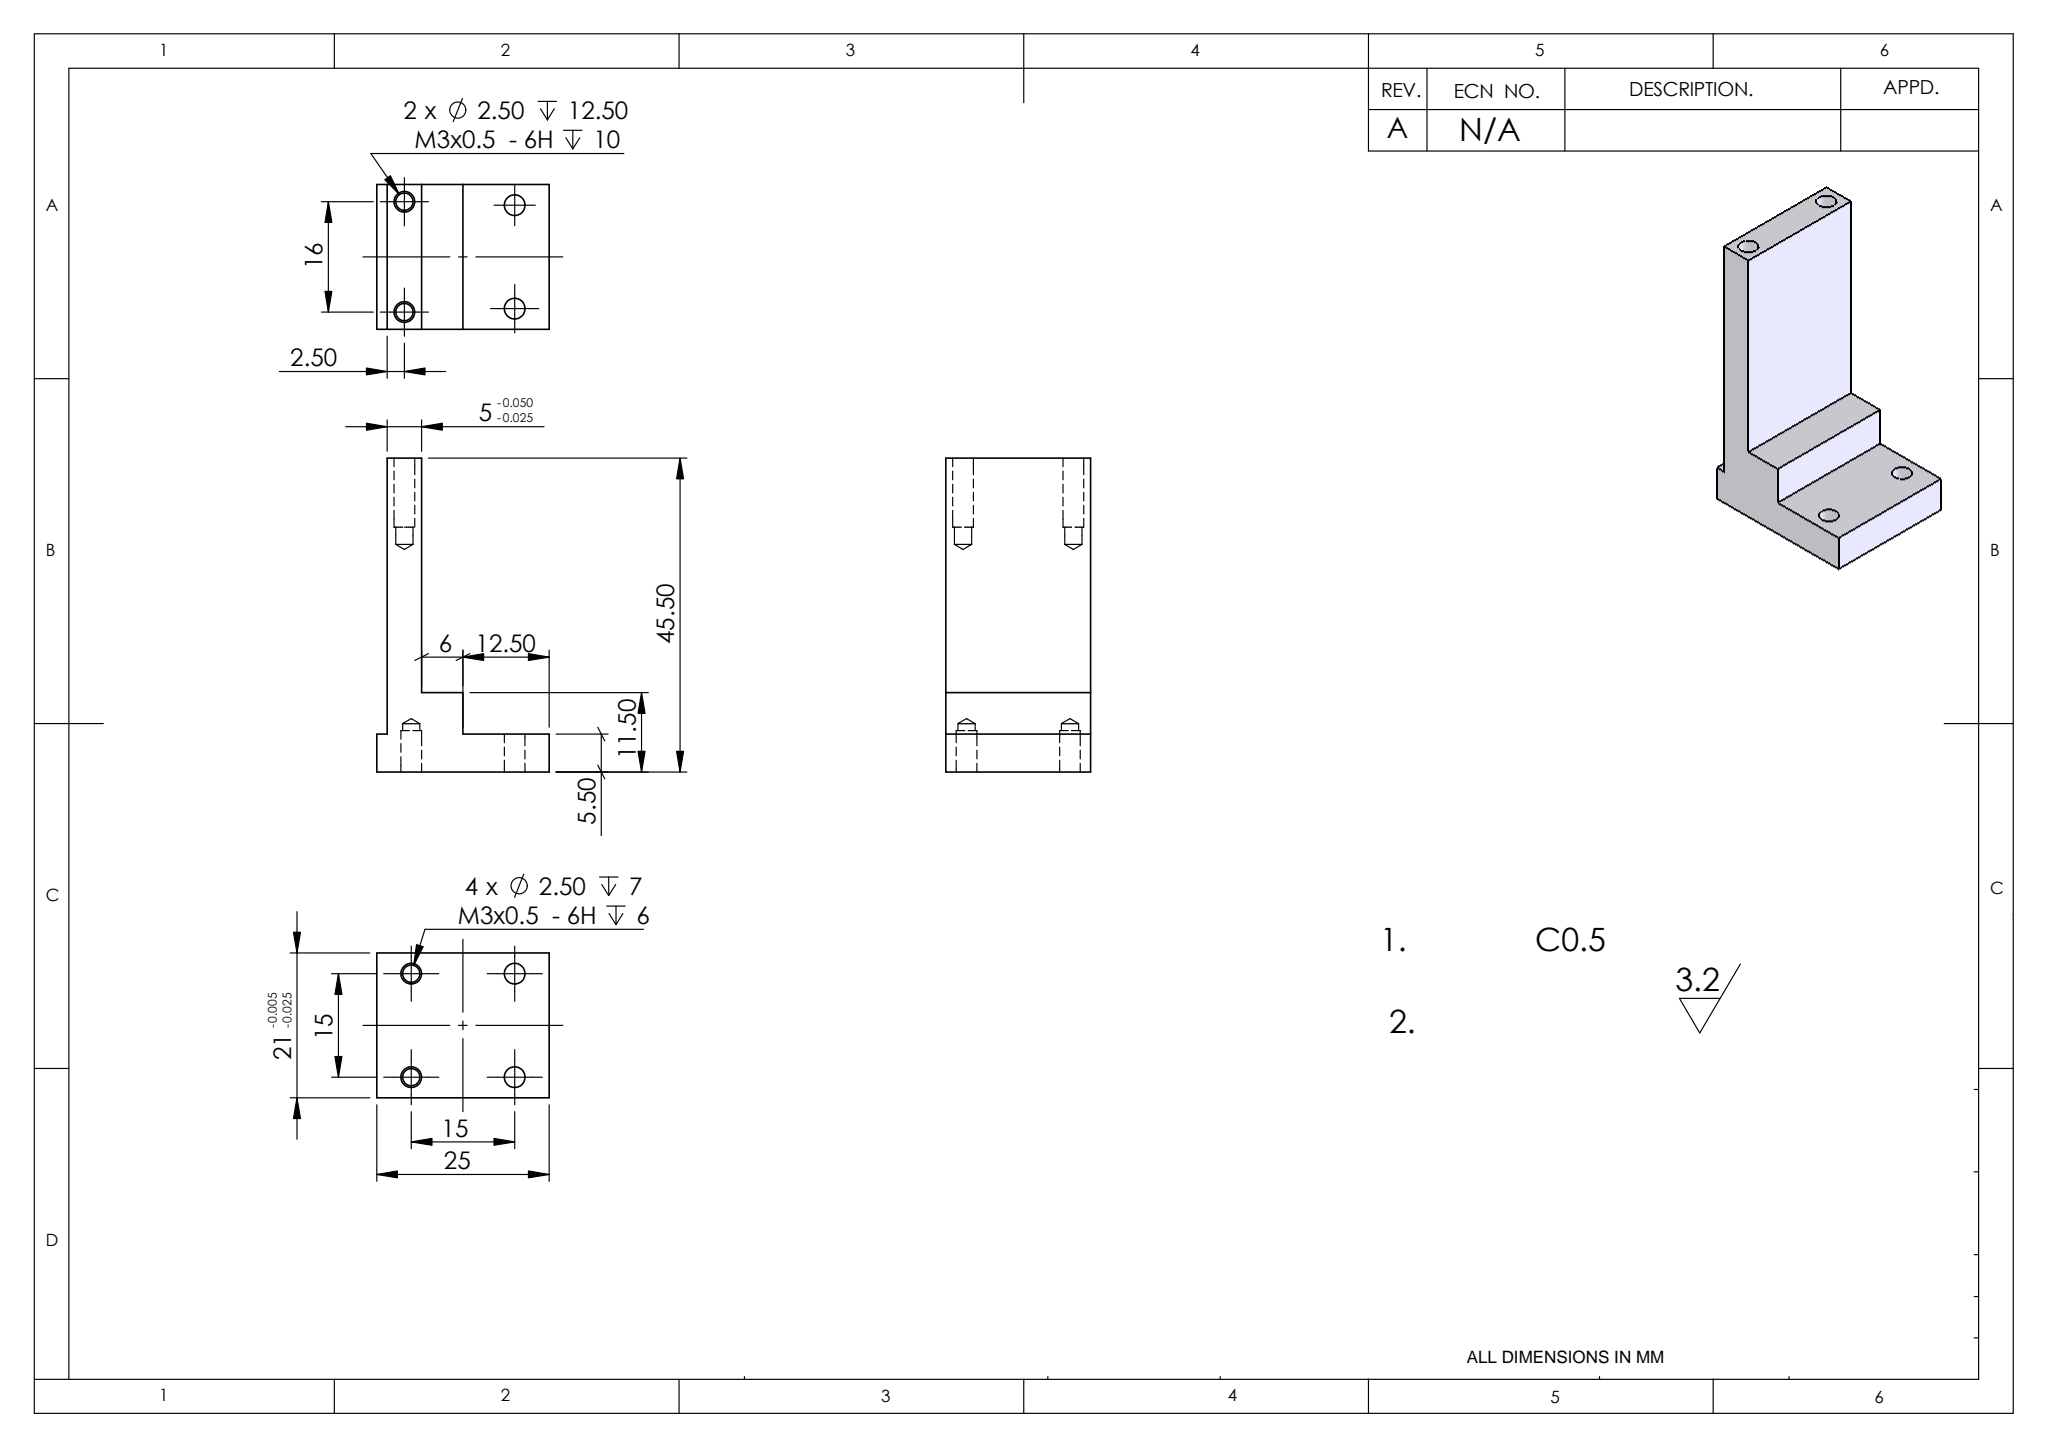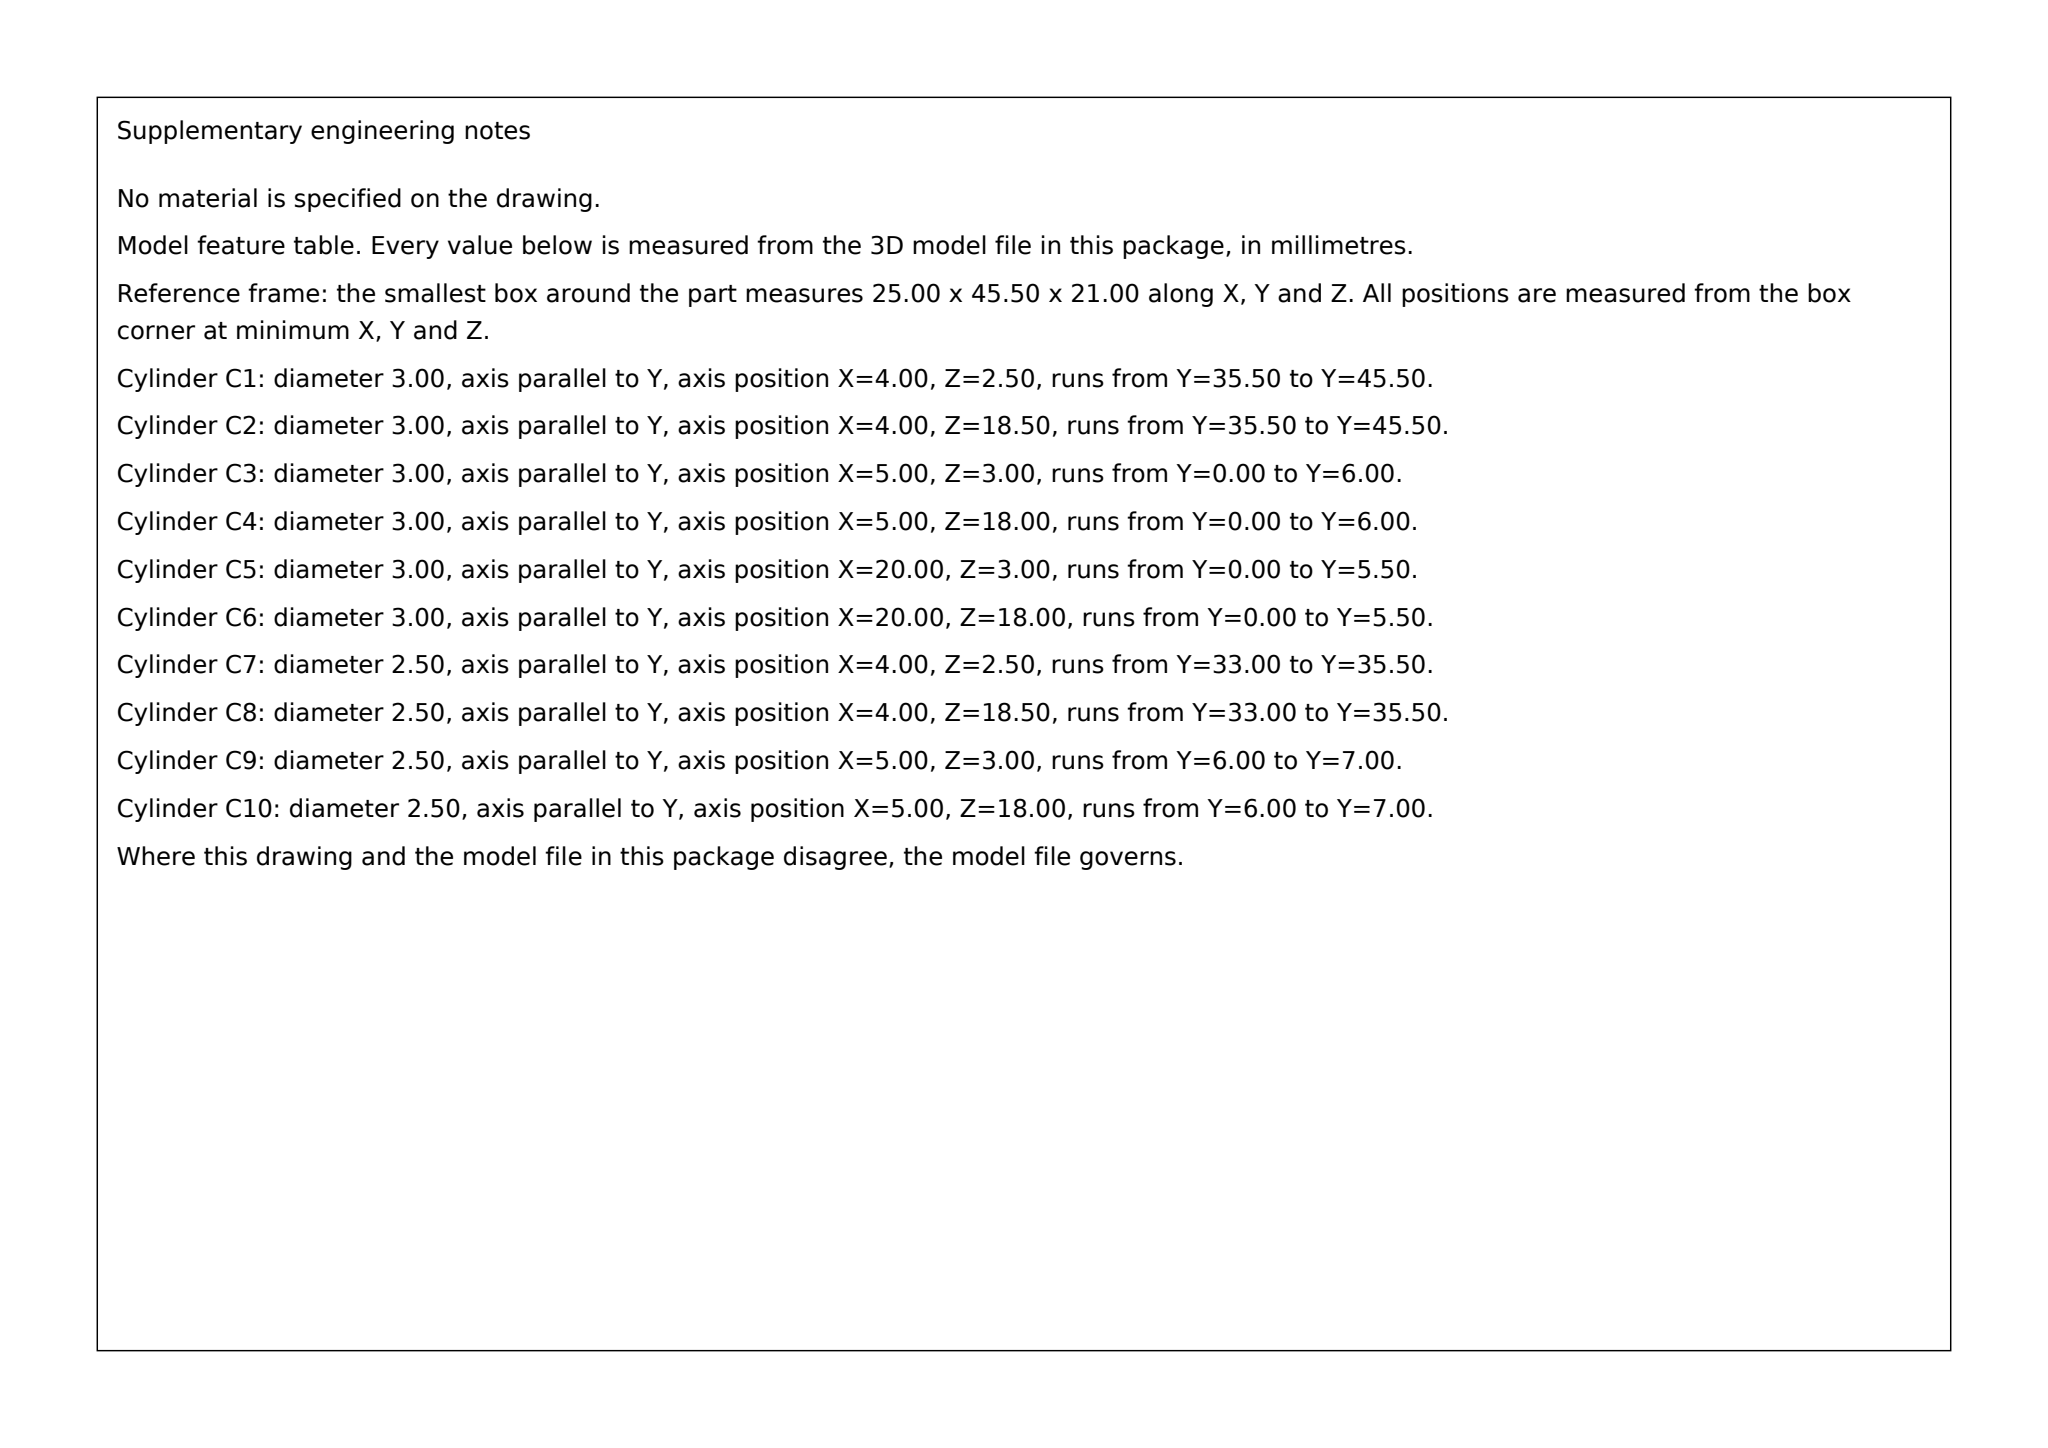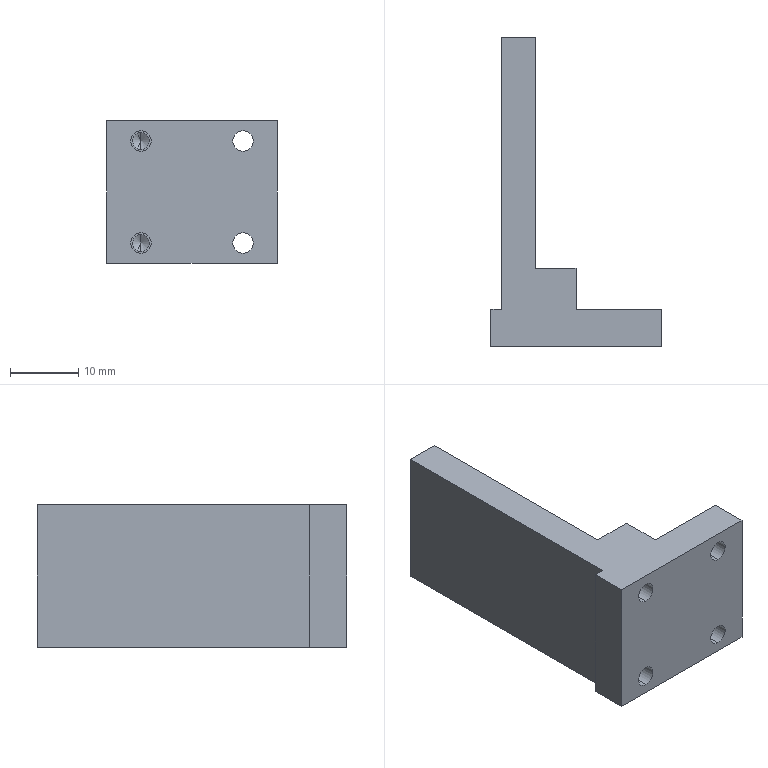Part | SolidWorks | mm | 1 solid | 44 faces | box 25 x 45.5 x 21 mm | volume 7500 mm3 | cylinder 20 | plane 16 | cone 8 | commonest cylinder face diameters 3 x12 2.5 x8
build123d program:
from build123d import *

# Parameters (mm, degrees)
SKETCH2_W                   = 21
SKETCH2_H                   = 40
EXTRUDE1_DEPTH              = 5
M3_TAPPED_HOLE1_D           = 2.5
M3_TAPPED_HOLE1_DEPTH       = 12.5
M3_TAPPED_HOLE1_CBORE_D     = 3
M3_TAPPED_HOLE1_CBORE_DEPTH = 10
M3_TAPPED_HOLE1_TIP         = 0.7511
SKETCH5_W                   = 25
SKETCH5_H                   = 21
EXTRUDE2_DEPTH              = 5.5
SKETCH8_W                   = 6
SKETCH8_H                   = 6
EXTRUDE3_DEPTH              = 21
M3_TAPPED_HOLE2_D           = 2.5
M3_TAPPED_HOLE2_DEPTH       = 7
M3_TAPPED_HOLE2_CBORE_D     = 3
M3_TAPPED_HOLE2_CBORE_DEPTH = 6
M3_TAPPED_HOLE2_TIP         = 0.7511


with BuildPart() as part:
    # Sketch2 → Extrude1 (new body)
    with BuildSketch(Plane(origin=(0, 0, 0), x_dir=(0, 0, -1), z_dir=(1, 0, 0))):
        with Locations((-10.5, 20)):
            Rectangle(SKETCH2_W, SKETCH2_H)
    extrude(amount=EXTRUDE1_DEPTH)

    # M3 Tapped Hole1
    with Locations(Plane(origin=(0, 40, 0), x_dir=(-1, 0, 0), z_dir=(0, 1, 0))):
        with Locations((-2.5, 18.5), (-2.5, 2.5)):
            CounterBoreHole(M3_TAPPED_HOLE1_D / 2, M3_TAPPED_HOLE1_CBORE_D / 2, M3_TAPPED_HOLE1_CBORE_DEPTH, depth=M3_TAPPED_HOLE1_DEPTH)
            with Locations((0, 0, -(M3_TAPPED_HOLE1_DEPTH + M3_TAPPED_HOLE1_TIP / 2))):  # 118° drill point
                Cone(0, M3_TAPPED_HOLE1_D / 2, M3_TAPPED_HOLE1_TIP, mode=Mode.SUBTRACT)

    # Sketch5 → Extrude2 (add)
    with BuildSketch(Plane.XZ):
        with Locations((11, 10.5)):
            Rectangle(SKETCH5_W, SKETCH5_H)
    extrude(amount=EXTRUDE2_DEPTH)

    # Sketch8 → Extrude3 (add)
    with BuildSketch(Plane.XY.offset(21)):
        with Locations((8, 3)):
            Rectangle(SKETCH8_W, SKETCH8_H)
    extrude(amount=-EXTRUDE3_DEPTH)

    # M3 Tapped Hole2
    with Locations(Plane(origin=(3.5, -5.5, 18), x_dir=(0, 0, -1), z_dir=(0, -1, 0))):
        with Locations((0, 0), (15, 0), (15, 15), (0, 15)):
            CounterBoreHole(M3_TAPPED_HOLE2_D / 2, M3_TAPPED_HOLE2_CBORE_D / 2, M3_TAPPED_HOLE2_CBORE_DEPTH, depth=M3_TAPPED_HOLE2_DEPTH)
            with Locations((0, 0, -(M3_TAPPED_HOLE2_DEPTH + M3_TAPPED_HOLE2_TIP / 2))):  # 118° drill point
                Cone(0, M3_TAPPED_HOLE2_D / 2, M3_TAPPED_HOLE2_TIP, mode=Mode.SUBTRACT)


solid = part.part